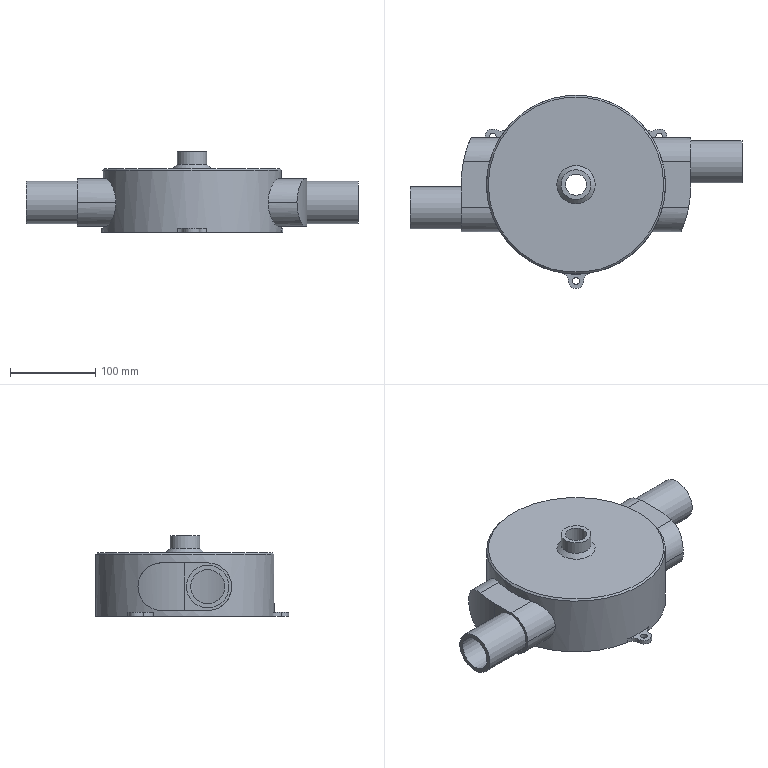Component | NX | PUMP_BODY | 1 solid | 65 faces | volume 571899 mm3 | cylinder 40 | plane 21 | cone 3 | torus 1 | commonest cylinder face diameters 56 x8 46 x8 20 x6 18 x3 8 x3 270 x2 50 x2 260 x2